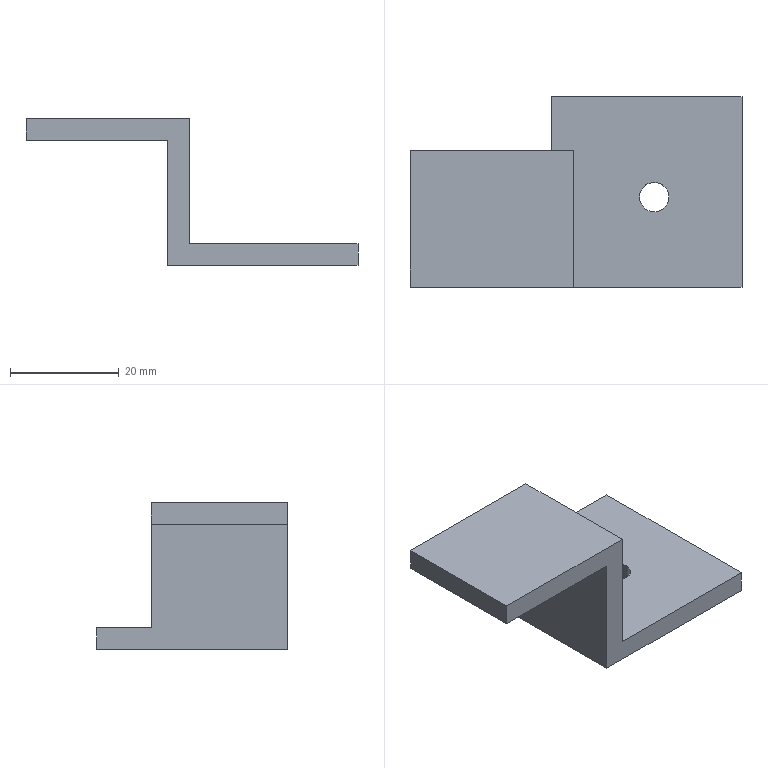Component | SolidWorks | LargeFunnelFixing-1 | 1 solid | 13 faces | box 61 x 35 x 27 mm | volume 9708 mm3 | plane 11 | cylinder 2 | commonest cylinder face diameters 5.4 x2
build123d program:
from build123d import *

# Parameters (mm, degrees)
BOSS_EXTRUDE1_DEPTH = 25
SKETCH3_R           = 2.7
CUT_EXTRUDE1_DEPTH  = 25
SKETCH5_W           = 35
SKETCH5_H           = 4
BOSS_EXTRUDE2_DEPTH = 10


with BuildPart() as part:
    # Sketch2 → Boss-Extrude1 (new body)
    with BuildSketch(Plane.XY):
        Polygon((-28.776, -10), (-58.776, -10), (-58.776, -33), (-89.776, -33), (-89.776, -37), (-54.776, -37), (-54.776, -14), (-28.776, -14), align=None)
    extrude(amount=-BOSS_EXTRUDE1_DEPTH)

    # Sketch3 → Cut-Extrude1 (cut)
    with BuildSketch(Plane(origin=(0, -33, 0), x_dir=(1, 0, 0), z_dir=(0, 1, 0))):
        with Locations(Location((-73.65, 8.438, 0), (0, 0, 180))):
            Circle(SKETCH3_R)
    extrude(amount=-CUT_EXTRUDE1_DEPTH, mode=Mode.SUBTRACT)

    # Sketch5 → Boss-Extrude2 (add)
    with BuildSketch(Plane.XY):
        with Locations((-72.276, -35)):
            Rectangle(SKETCH5_W, SKETCH5_H)
    extrude(amount=BOSS_EXTRUDE2_DEPTH)


solid = part.part

# Placed as in the assembly
solid = solid.moved(Location((-624.146, 60.55, 354.126), (-90, 0, 180)))
STEP:
#1=COLOUR_RGB('',0.7922,0.8196,0.9333);
#2=FILL_AREA_STYLE_COLOUR('',#1);
#3=FILL_AREA_STYLE('',(#2));
#4=SURFACE_STYLE_FILL_AREA(#3);
#5=SURFACE_SIDE_STYLE('',(#4));
#6=SURFACE_STYLE_USAGE(.BOTH.,#5);
#7=PRESENTATION_STYLE_ASSIGNMENT((#6));
#8=CARTESIAN_POINT('',(-21.567,2.052,12.485));
#9=VERTEX_POINT('',#8);
#10=CARTESIAN_POINT('',(-21.779,2.052,12.485));
#11=VERTEX_POINT('',#10);
#12=CARTESIAN_POINT('',(-21.673,2.052,12.485));
#13=DIRECTION('',(-0.,0.,-1.));
#14=DIRECTION('',(-1.,0.,0.));
#15=AXIS2_PLACEMENT_3D('',#12,#13,#14);
#16=CIRCLE('',#15,0.1063);
#17=EDGE_CURVE('',#9,#11,#16,.T.);
#18=ORIENTED_EDGE('',*,*,#17,.T.);
#19=CARTESIAN_POINT('',(-21.779,2.052,12.643));
#20=VERTEX_POINT('',#19);
#21=CARTESIAN_POINT('',(-21.779,2.052,11.658));
#22=DIRECTION('',(0.,-0.,1.));
#23=VECTOR('',#22,39.37);
#24=LINE('',#21,#23);
#25=EDGE_CURVE('',#11,#20,#24,.T.);
#26=ORIENTED_EDGE('',*,*,#25,.T.);
#27=CARTESIAN_POINT('',(-21.567,2.052,12.643));
#28=VERTEX_POINT('',#27);
#29=CARTESIAN_POINT('',(-21.673,2.052,12.643));
#30=DIRECTION('',(0.,-0.,1.));
#31=DIRECTION('',(1.,0.,0.));
#32=AXIS2_PLACEMENT_3D('',#29,#30,#31);
#33=CIRCLE('',#32,0.1063);
#34=EDGE_CURVE('',#20,#28,#33,.T.);
#35=ORIENTED_EDGE('',*,*,#34,.T.);
#36=CARTESIAN_POINT('',(-21.567,2.052,11.658));
#37=DIRECTION('',(0.,-0.,1.));
#38=VECTOR('',#37,39.37);
#39=LINE('',#36,#38);
#40=EDGE_CURVE('',#9,#28,#39,.T.);
#41=ORIENTED_EDGE('',*,*,#40,.F.);
#42=EDGE_LOOP('',(#18,#26,#35,#41));
#43=FACE_OUTER_BOUND('',#42,.T.);
#44=CARTESIAN_POINT('',(-21.673,2.052,11.658));
#45=DIRECTION('',(0.,-0.,1.));
#46=DIRECTION('',(1.,0.,0.));
#47=AXIS2_PLACEMENT_3D('',#44,#45,#46);
#48=CYLINDRICAL_SURFACE('',#47,0.1063);
#49=ADVANCED_FACE('',(#43),#48,.F.);
#50=CARTESIAN_POINT('',(-22.416,2.384,12.643));
#51=VERTEX_POINT('',#50);
#52=CARTESIAN_POINT('',(-22.259,2.384,12.643));
#53=VERTEX_POINT('',#52);
#54=CARTESIAN_POINT('',(-21.038,2.384,12.643));
#55=DIRECTION('',(1.,-0.,0.));
#56=VECTOR('',#55,39.37);
#57=LINE('',#54,#56);
#58=EDGE_CURVE('',#51,#53,#57,.T.);
#59=ORIENTED_EDGE('',*,*,#58,.F.);
#60=CARTESIAN_POINT('',(-22.416,2.384,13.391));
#61=VERTEX_POINT('',#60);
#62=CARTESIAN_POINT('',(-22.416,2.384,13.391));
#63=DIRECTION('',(-0.,-0.,1.));
#64=VECTOR('',#63,39.37);
#65=LINE('',#62,#64);
#66=EDGE_CURVE('',#51,#61,#65,.T.);
#67=ORIENTED_EDGE('',*,*,#66,.T.);
#68=CARTESIAN_POINT('',(-23.44,2.384,13.391));
#69=VERTEX_POINT('',#68);
#70=CARTESIAN_POINT('',(-23.44,2.384,13.391));
#71=DIRECTION('',(-1.,0.,0.));
#72=VECTOR('',#71,39.37);
#73=LINE('',#70,#72);
#74=EDGE_CURVE('',#61,#69,#73,.T.);
#75=ORIENTED_EDGE('',*,*,#74,.T.);
#76=CARTESIAN_POINT('',(-23.44,2.384,13.548));
#77=VERTEX_POINT('',#76);
#78=CARTESIAN_POINT('',(-23.44,2.384,13.548));
#79=DIRECTION('',(-0.,-0.,1.));
#80=VECTOR('',#79,39.37);
#81=LINE('',#78,#80);
#82=EDGE_CURVE('',#69,#77,#81,.T.);
#83=ORIENTED_EDGE('',*,*,#82,.T.);
#84=CARTESIAN_POINT('',(-22.259,2.384,13.548));
#85=VERTEX_POINT('',#84);
#86=CARTESIAN_POINT('',(-23.44,2.384,13.548));
#87=DIRECTION('',(1.,-0.,-0.));
#88=VECTOR('',#87,39.37);
#89=LINE('',#86,#88);
#90=EDGE_CURVE('',#77,#85,#89,.T.);
#91=ORIENTED_EDGE('',*,*,#90,.T.);
#92=CARTESIAN_POINT('',(-22.259,2.384,13.548));
#93=DIRECTION('',(0.,0.,-1.));
#94=VECTOR('',#93,39.37);
#95=LINE('',#92,#94);
#96=EDGE_CURVE('',#85,#53,#95,.T.);
#97=ORIENTED_EDGE('',*,*,#96,.T.);
#98=EDGE_LOOP('',(#59,#67,#75,#83,#91,#97));
#99=FACE_OUTER_BOUND('',#98,.T.);
#100=CARTESIAN_POINT('',(-24.573,2.384,13.942));
#101=DIRECTION('',(-0.,-1.,-0.));
#102=DIRECTION('',(1.,-0.,0.));
#103=AXIS2_PLACEMENT_3D('',#100,#101,#102);
#104=PLANE('',#103);
#105=ADVANCED_FACE('',(#99),#104,.F.);
#106=ORIENTED_EDGE('',*,*,#82,.F.);
#107=CARTESIAN_POINT('',(-23.44,1.4,13.391));
#108=VERTEX_POINT('',#107);
#109=CARTESIAN_POINT('',(-23.44,1.4,13.391));
#110=DIRECTION('',(0.,1.,0.));
#111=VECTOR('',#110,39.37);
#112=LINE('',#109,#111);
#113=EDGE_CURVE('',#108,#69,#112,.T.);
#114=ORIENTED_EDGE('',*,*,#113,.F.);
#115=CARTESIAN_POINT('',(-23.44,1.4,13.548));
#116=VERTEX_POINT('',#115);
#117=CARTESIAN_POINT('',(-23.44,1.4,13.548));
#118=DIRECTION('',(-0.,-0.,1.));
#119=VECTOR('',#118,39.37);
#120=LINE('',#117,#119);
#121=EDGE_CURVE('',#108,#116,#120,.T.);
#122=ORIENTED_EDGE('',*,*,#121,.T.);
#123=CARTESIAN_POINT('',(-23.44,1.4,13.548));
#124=DIRECTION('',(0.,1.,0.));
#125=VECTOR('',#124,39.37);
#126=LINE('',#123,#125);
#127=EDGE_CURVE('',#116,#77,#126,.T.);
#128=ORIENTED_EDGE('',*,*,#127,.T.);
#129=EDGE_LOOP('',(#106,#114,#122,#128));
#130=FACE_OUTER_BOUND('',#129,.T.);
#131=CARTESIAN_POINT('',(-23.44,1.4,13.548));
#132=DIRECTION('',(-1.,0.,-0.));
#133=DIRECTION('',(-0.,-1.,-0.));
#134=AXIS2_PLACEMENT_3D('',#131,#132,#133);
#135=PLANE('',#134);
#136=ADVANCED_FACE('',(#130),#135,.T.);
#137=ORIENTED_EDGE('',*,*,#74,.F.);
#138=CARTESIAN_POINT('',(-22.416,1.4,13.391));
#139=VERTEX_POINT('',#138);
#140=CARTESIAN_POINT('',(-22.416,1.4,13.391));
#141=DIRECTION('',(0.,1.,0.));
#142=VECTOR('',#141,39.37);
#143=LINE('',#140,#142);
#144=EDGE_CURVE('',#139,#61,#143,.T.);
#145=ORIENTED_EDGE('',*,*,#144,.F.);
#146=CARTESIAN_POINT('',(-23.44,1.4,13.391));
#147=DIRECTION('',(-1.,0.,0.));
#148=VECTOR('',#147,39.37);
#149=LINE('',#146,#148);
#150=EDGE_CURVE('',#139,#108,#149,.T.);
#151=ORIENTED_EDGE('',*,*,#150,.T.);
#152=ORIENTED_EDGE('',*,*,#113,.T.);
#153=EDGE_LOOP('',(#137,#145,#151,#152));
#154=FACE_OUTER_BOUND('',#153,.T.);
#155=CARTESIAN_POINT('',(-23.44,1.4,13.391));
#156=DIRECTION('',(-0.,0.,-1.));
#157=DIRECTION('',(-1.,0.,0.));
#158=AXIS2_PLACEMENT_3D('',#155,#156,#157);
#159=PLANE('',#158);
#160=ADVANCED_FACE('',(#154),#159,.T.);
#161=ORIENTED_EDGE('',*,*,#66,.F.);
#162=CARTESIAN_POINT('',(-22.416,2.778,12.643));
#163=VERTEX_POINT('',#162);
#164=CARTESIAN_POINT('',(-22.416,2.778,12.643));
#165=DIRECTION('',(-0.,-1.,-0.));
#166=VECTOR('',#165,39.37);
#167=LINE('',#164,#166);
#168=EDGE_CURVE('',#163,#51,#167,.T.);
#169=ORIENTED_EDGE('',*,*,#168,.F.);
#170=CARTESIAN_POINT('',(-22.416,2.778,12.485));
#171=VERTEX_POINT('',#170);
#172=CARTESIAN_POINT('',(-22.416,2.778,12.643));
#173=DIRECTION('',(-0.,-0.,1.));
#174=VECTOR('',#173,39.37);
#175=LINE('',#172,#174);
#176=EDGE_CURVE('',#171,#163,#175,.T.);
#177=ORIENTED_EDGE('',*,*,#176,.F.);
#178=CARTESIAN_POINT('',(-22.416,1.4,12.485));
#179=VERTEX_POINT('',#178);
#180=CARTESIAN_POINT('',(-22.416,1.4,12.485));
#181=DIRECTION('',(0.,1.,0.));
#182=VECTOR('',#181,39.37);
#183=LINE('',#180,#182);
#184=EDGE_CURVE('',#179,#171,#183,.T.);
#185=ORIENTED_EDGE('',*,*,#184,.F.);
#186=CARTESIAN_POINT('',(-22.416,1.4,13.391));
#187=DIRECTION('',(-0.,-0.,1.));
#188=VECTOR('',#187,39.37);
#189=LINE('',#186,#188);
#190=EDGE_CURVE('',#179,#139,#189,.T.);
#191=ORIENTED_EDGE('',*,*,#190,.T.);
#192=ORIENTED_EDGE('',*,*,#144,.T.);
#193=EDGE_LOOP('',(#161,#169,#177,#185,#191,#192));
#194=FACE_OUTER_BOUND('',#193,.T.);
#195=CARTESIAN_POINT('',(-22.416,1.4,13.391));
#196=DIRECTION('',(-1.,0.,-0.));
#197=DIRECTION('',(-0.,-1.,-0.));
#198=AXIS2_PLACEMENT_3D('',#195,#196,#197);
#199=PLANE('',#198);
#200=ADVANCED_FACE('',(#194),#199,.T.);
#201=ORIENTED_EDGE('',*,*,#17,.F.);
#202=CARTESIAN_POINT('',(-21.673,2.052,12.485));
#203=DIRECTION('',(-0.,0.,-1.));
#204=DIRECTION('',(-1.,0.,0.));
#205=AXIS2_PLACEMENT_3D('',#202,#203,#204);
#206=CIRCLE('',#205,0.1063);
#207=EDGE_CURVE('',#11,#9,#206,.T.);
#208=ORIENTED_EDGE('',*,*,#207,.F.);
#209=EDGE_LOOP('',(#201,#208));
#210=FACE_BOUND('',#209,.T.);
#211=ORIENTED_EDGE('',*,*,#184,.T.);
#212=CARTESIAN_POINT('',(-21.038,2.778,12.485));
#213=VERTEX_POINT('',#212);
#214=CARTESIAN_POINT('',(-21.038,2.778,12.485));
#215=DIRECTION('',(-1.,0.,-0.));
#216=VECTOR('',#215,39.37);
#217=LINE('',#214,#216);
#218=EDGE_CURVE('',#213,#171,#217,.T.);
#219=ORIENTED_EDGE('',*,*,#218,.F.);
#220=CARTESIAN_POINT('',(-21.038,1.4,12.485));
#221=VERTEX_POINT('',#220);
#222=CARTESIAN_POINT('',(-21.038,1.4,12.485));
#223=DIRECTION('',(0.,1.,0.));
#224=VECTOR('',#223,39.37);
#225=LINE('',#222,#224);
#226=EDGE_CURVE('',#221,#213,#225,.T.);
#227=ORIENTED_EDGE('',*,*,#226,.F.);
#228=CARTESIAN_POINT('',(-22.416,1.4,12.485));
#229=DIRECTION('',(-1.,0.,0.));
#230=VECTOR('',#229,39.37);
#231=LINE('',#228,#230);
#232=EDGE_CURVE('',#221,#179,#231,.T.);
#233=ORIENTED_EDGE('',*,*,#232,.T.);
#234=EDGE_LOOP('',(#211,#219,#227,#233));
#235=FACE_OUTER_BOUND('',#234,.T.);
#236=CARTESIAN_POINT('',(-22.416,1.4,12.485));
#237=DIRECTION('',(-0.,0.,-1.));
#238=DIRECTION('',(-1.,0.,0.));
#239=AXIS2_PLACEMENT_3D('',#236,#237,#238);
#240=PLANE('',#239);
#241=ADVANCED_FACE('',(#210,#235),#240,.T.);
#242=ORIENTED_EDGE('',*,*,#226,.T.);
#243=CARTESIAN_POINT('',(-21.038,2.778,12.643));
#244=VERTEX_POINT('',#243);
#245=CARTESIAN_POINT('',(-21.038,2.778,12.643));
#246=DIRECTION('',(0.,0.,-1.));
#247=VECTOR('',#246,39.37);
#248=LINE('',#245,#247);
#249=EDGE_CURVE('',#244,#213,#248,.T.);
#250=ORIENTED_EDGE('',*,*,#249,.F.);
#251=CARTESIAN_POINT('',(-21.038,1.4,12.643));
#252=VERTEX_POINT('',#251);
#253=CARTESIAN_POINT('',(-21.038,1.4,12.643));
#254=DIRECTION('',(0.,1.,0.));
#255=VECTOR('',#254,39.37);
#256=LINE('',#253,#255);
#257=EDGE_CURVE('',#252,#244,#256,.T.);
#258=ORIENTED_EDGE('',*,*,#257,.F.);
#259=CARTESIAN_POINT('',(-21.038,1.4,12.485));
#260=DIRECTION('',(0.,0.,-1.));
#261=VECTOR('',#260,39.37);
#262=LINE('',#259,#261);
#263=EDGE_CURVE('',#252,#221,#262,.T.);
#264=ORIENTED_EDGE('',*,*,#263,.T.);
#265=EDGE_LOOP('',(#242,#250,#258,#264));
#266=FACE_OUTER_BOUND('',#265,.T.);
#267=CARTESIAN_POINT('',(-21.038,1.4,12.485));
#268=DIRECTION('',(1.,-0.,0.));
#269=DIRECTION('',(0.,1.,0.));
#270=AXIS2_PLACEMENT_3D('',#267,#268,#269);
#271=PLANE('',#270);
#272=ADVANCED_FACE('',(#266),#271,.T.);
#273=CARTESIAN_POINT('',(-21.673,2.052,12.643));
#274=DIRECTION('',(0.,-0.,1.));
#275=DIRECTION('',(1.,0.,0.));
#276=AXIS2_PLACEMENT_3D('',#273,#274,#275);
#277=CIRCLE('',#276,0.1063);
#278=EDGE_CURVE('',#28,#20,#277,.T.);
#279=ORIENTED_EDGE('',*,*,#278,.F.);
#280=ORIENTED_EDGE('',*,*,#34,.F.);
#281=EDGE_LOOP('',(#279,#280));
#282=FACE_BOUND('',#281,.T.);
#283=ORIENTED_EDGE('',*,*,#257,.T.);
#284=CARTESIAN_POINT('',(-21.038,2.778,12.643));
#285=DIRECTION('',(1.,-0.,0.));
#286=VECTOR('',#285,39.37);
#287=LINE('',#284,#286);
#288=EDGE_CURVE('',#163,#244,#287,.T.);
#289=ORIENTED_EDGE('',*,*,#288,.F.);
#290=ORIENTED_EDGE('',*,*,#168,.T.);
#291=ORIENTED_EDGE('',*,*,#58,.T.);
#292=CARTESIAN_POINT('',(-22.259,1.4,12.643));
#293=VERTEX_POINT('',#292);
#294=CARTESIAN_POINT('',(-22.259,1.4,12.643));
#295=DIRECTION('',(0.,1.,0.));
#296=VECTOR('',#295,39.37);
#297=LINE('',#294,#296);
#298=EDGE_CURVE('',#293,#53,#297,.T.);
#299=ORIENTED_EDGE('',*,*,#298,.F.);
#300=CARTESIAN_POINT('',(-22.259,1.4,12.643));
#301=DIRECTION('',(1.,-0.,-0.));
#302=VECTOR('',#301,39.37);
#303=LINE('',#300,#302);
#304=EDGE_CURVE('',#293,#252,#303,.T.);
#305=ORIENTED_EDGE('',*,*,#304,.T.);
#306=EDGE_LOOP('',(#283,#289,#290,#291,#299,#305));
#307=FACE_OUTER_BOUND('',#306,.T.);
#308=CARTESIAN_POINT('',(-22.259,1.4,12.643));
#309=DIRECTION('',(0.,-0.,1.));
#310=DIRECTION('',(1.,-0.,-0.));
#311=AXIS2_PLACEMENT_3D('',#308,#309,#310);
#312=PLANE('',#311);
#313=ADVANCED_FACE('',(#282,#307),#312,.T.);
#314=ORIENTED_EDGE('',*,*,#96,.F.);
#315=CARTESIAN_POINT('',(-22.259,1.4,13.548));
#316=VERTEX_POINT('',#315);
#317=CARTESIAN_POINT('',(-22.259,1.4,13.548));
#318=DIRECTION('',(0.,1.,0.));
#319=VECTOR('',#318,39.37);
#320=LINE('',#317,#319);
#321=EDGE_CURVE('',#316,#85,#320,.T.);
#322=ORIENTED_EDGE('',*,*,#321,.F.);
#323=CARTESIAN_POINT('',(-22.259,1.4,13.548));
#324=DIRECTION('',(0.,0.,-1.));
#325=VECTOR('',#324,39.37);
#326=LINE('',#323,#325);
#327=EDGE_CURVE('',#316,#293,#326,.T.);
#328=ORIENTED_EDGE('',*,*,#327,.T.);
#329=ORIENTED_EDGE('',*,*,#298,.T.);
#330=EDGE_LOOP('',(#314,#322,#328,#329));
#331=FACE_OUTER_BOUND('',#330,.T.);
#332=CARTESIAN_POINT('',(-22.259,1.4,13.548));
#333=DIRECTION('',(1.,-0.,0.));
#334=DIRECTION('',(0.,0.,-1.));
#335=AXIS2_PLACEMENT_3D('',#332,#333,#334);
#336=PLANE('',#335);
#337=ADVANCED_FACE('',(#331),#336,.T.);
#338=ORIENTED_EDGE('',*,*,#90,.F.);
#339=ORIENTED_EDGE('',*,*,#127,.F.);
#340=CARTESIAN_POINT('',(-23.44,1.4,13.548));
#341=DIRECTION('',(1.,-0.,-0.));
#342=VECTOR('',#341,39.37);
#343=LINE('',#340,#342);
#344=EDGE_CURVE('',#116,#316,#343,.T.);
#345=ORIENTED_EDGE('',*,*,#344,.T.);
#346=ORIENTED_EDGE('',*,*,#321,.T.);
#347=EDGE_LOOP('',(#338,#339,#345,#346));
#348=FACE_OUTER_BOUND('',#347,.T.);
#349=CARTESIAN_POINT('',(-23.44,1.4,13.548));
#350=DIRECTION('',(0.,-0.,1.));
#351=DIRECTION('',(1.,-0.,-0.));
#352=AXIS2_PLACEMENT_3D('',#349,#350,#351);
#353=PLANE('',#352);
#354=ADVANCED_FACE('',(#348),#353,.T.);
#355=ORIENTED_EDGE('',*,*,#121,.F.);
#356=ORIENTED_EDGE('',*,*,#150,.F.);
#357=ORIENTED_EDGE('',*,*,#190,.F.);
#358=ORIENTED_EDGE('',*,*,#232,.F.);
#359=ORIENTED_EDGE('',*,*,#263,.F.);
#360=ORIENTED_EDGE('',*,*,#304,.F.);
#361=ORIENTED_EDGE('',*,*,#327,.F.);
#362=ORIENTED_EDGE('',*,*,#344,.F.);
#363=EDGE_LOOP('',(#355,#356,#357,#358,#359,#360,#361,#362));
#364=FACE_OUTER_BOUND('',#363,.T.);
#365=CARTESIAN_POINT('',(-24.573,1.4,13.942));
#366=DIRECTION('',(-0.,-1.,-0.));
#367=DIRECTION('',(1.,-0.,0.));
#368=AXIS2_PLACEMENT_3D('',#365,#366,#367);
#369=PLANE('',#368);
#370=ADVANCED_FACE('',(#364),#369,.T.);
#371=ORIENTED_EDGE('',*,*,#25,.F.);
#372=ORIENTED_EDGE('',*,*,#207,.T.);
#373=ORIENTED_EDGE('',*,*,#40,.T.);
#374=ORIENTED_EDGE('',*,*,#278,.T.);
#375=EDGE_LOOP('',(#371,#372,#373,#374));
#376=FACE_OUTER_BOUND('',#375,.T.);
#377=CARTESIAN_POINT('',(-21.673,2.052,11.658));
#378=DIRECTION('',(0.,-0.,1.));
#379=DIRECTION('',(1.,0.,0.));
#380=AXIS2_PLACEMENT_3D('',#377,#378,#379);
#381=CYLINDRICAL_SURFACE('',#380,0.1063);
#382=ADVANCED_FACE('',(#376),#381,.F.);
#383=ORIENTED_EDGE('',*,*,#249,.T.);
#384=ORIENTED_EDGE('',*,*,#218,.T.);
#385=ORIENTED_EDGE('',*,*,#176,.T.);
#386=ORIENTED_EDGE('',*,*,#288,.T.);
#387=EDGE_LOOP('',(#383,#384,#385,#386));
#388=FACE_OUTER_BOUND('',#387,.T.);
#389=CARTESIAN_POINT('',(-24.573,2.778,13.942));
#390=DIRECTION('',(0.,1.,0.));
#391=DIRECTION('',(-1.,0.,-0.));
#392=AXIS2_PLACEMENT_3D('',#389,#390,#391);
#393=PLANE('',#392);
#394=ADVANCED_FACE('',(#388),#393,.T.);
#395=CLOSED_SHELL('',(#49,#105,#136,#160,#200,#241,#272,#313,#337,#354,#370,#382,#394));
#396=MANIFOLD_SOLID_BREP('',#395);
#397=STYLED_ITEM('',(#7),#396);
#398=(LENGTH_UNIT()NAMED_UNIT(*)SI_UNIT($,.METRE.));
#399=LENGTH_MEASURE_WITH_UNIT(LENGTH_MEASURE(0.0254),#398);
#400=DIMENSIONAL_EXPONENTS(1.,0.,0.,0.,0.,0.,0.);
#401=(CONVERSION_BASED_UNIT('',#399)LENGTH_UNIT()NAMED_UNIT(#400));
#402=UNCERTAINTY_MEASURE_WITH_UNIT(LENGTH_MEASURE(0.00001),#401,'','');
#403=(NAMED_UNIT(*)PLANE_ANGLE_UNIT()SI_UNIT($,.RADIAN.));
#404=(NAMED_UNIT(*)SI_UNIT($,.STERADIAN.)SOLID_ANGLE_UNIT());
#405=(GEOMETRIC_REPRESENTATION_CONTEXT(3)GLOBAL_UNCERTAINTY_ASSIGNED_CONTEXT((#402))GLOBAL_UNIT_ASSIGNED_CONTEXT((#401,#403,#404))REPRESENTATION_CONTEXT('',''));
#406=MECHANICAL_DESIGN_GEOMETRIC_PRESENTATION_REPRESENTATION('',(#397),#405);
#407=PRESENTATION_LAYER_ASSIGNMENT('','',(#397));
#408=CARTESIAN_POINT('',(0.,0.,0.));
#409=DIRECTION('',(0.,0.,1.));
#410=DIRECTION('',(1.,0.,0.));
#411=AXIS2_PLACEMENT_3D('',#408,#409,#410);
#412=(LENGTH_UNIT()NAMED_UNIT(*)SI_UNIT($,.METRE.));
#413=LENGTH_MEASURE_WITH_UNIT(LENGTH_MEASURE(0.0254),#412);
#414=DIMENSIONAL_EXPONENTS(1.,0.,0.,0.,0.,0.,0.);
#415=(CONVERSION_BASED_UNIT('',#413)LENGTH_UNIT()NAMED_UNIT(#414));
#416=UNCERTAINTY_MEASURE_WITH_UNIT(LENGTH_MEASURE(0.00001),#415,'','');
#417=(NAMED_UNIT(*)PLANE_ANGLE_UNIT()SI_UNIT($,.RADIAN.));
#418=(NAMED_UNIT(*)SI_UNIT($,.STERADIAN.)SOLID_ANGLE_UNIT());
#419=(GEOMETRIC_REPRESENTATION_CONTEXT(3)GLOBAL_UNCERTAINTY_ASSIGNED_CONTEXT((#416))GLOBAL_UNIT_ASSIGNED_CONTEXT((#415,#417,#418))REPRESENTATION_CONTEXT('',''));
#420=ADVANCED_BREP_SHAPE_REPRESENTATION('',(#396,#411),#419);